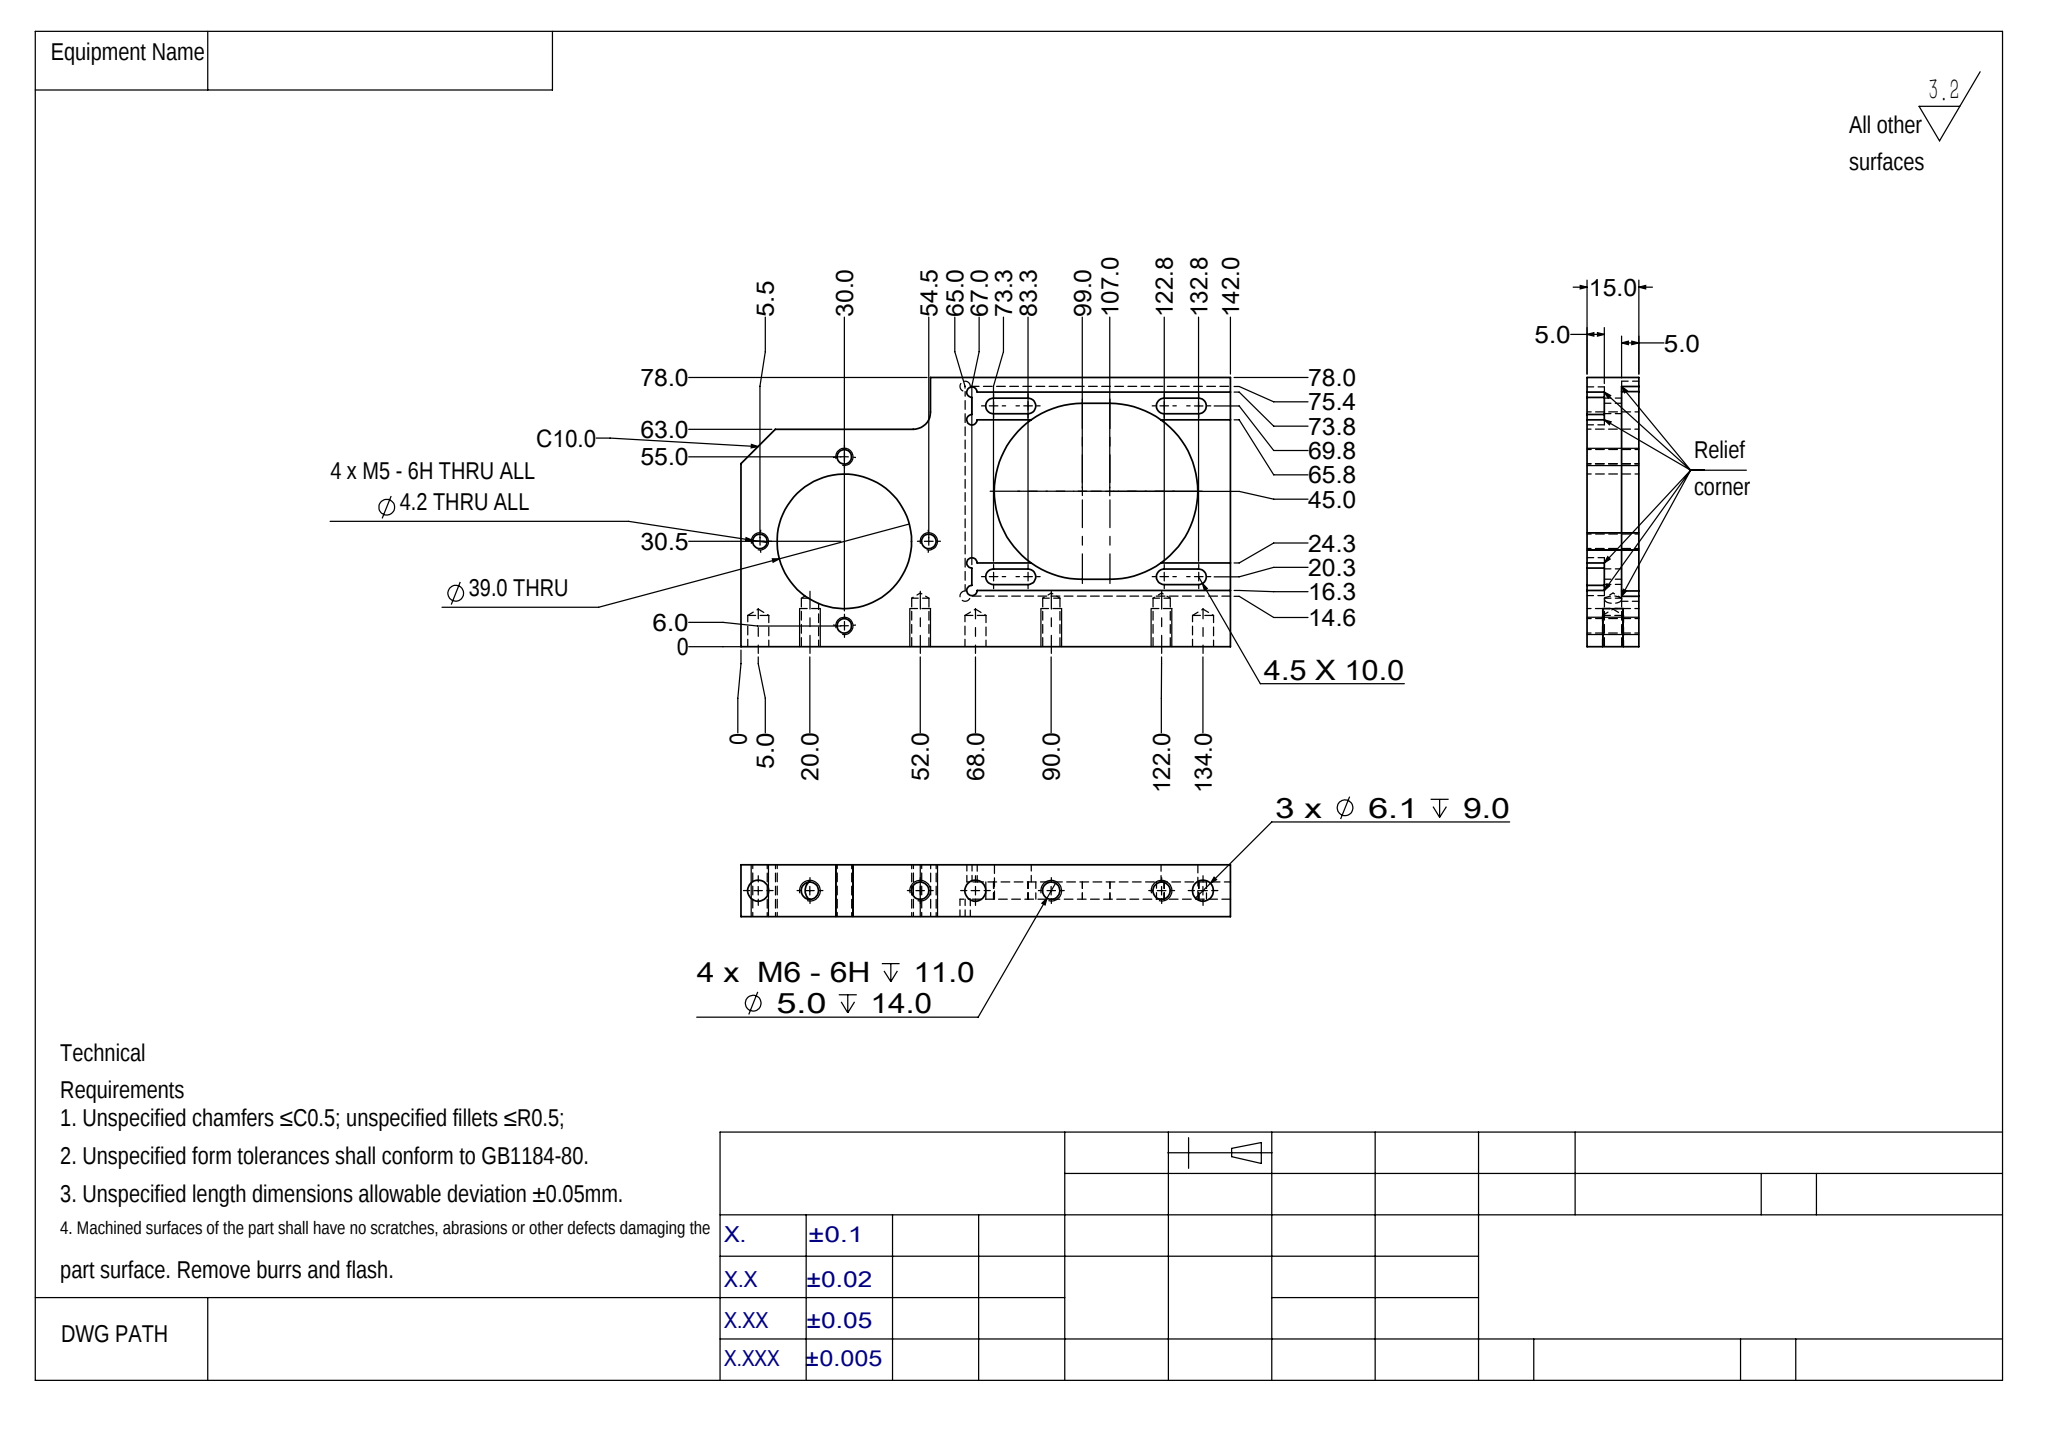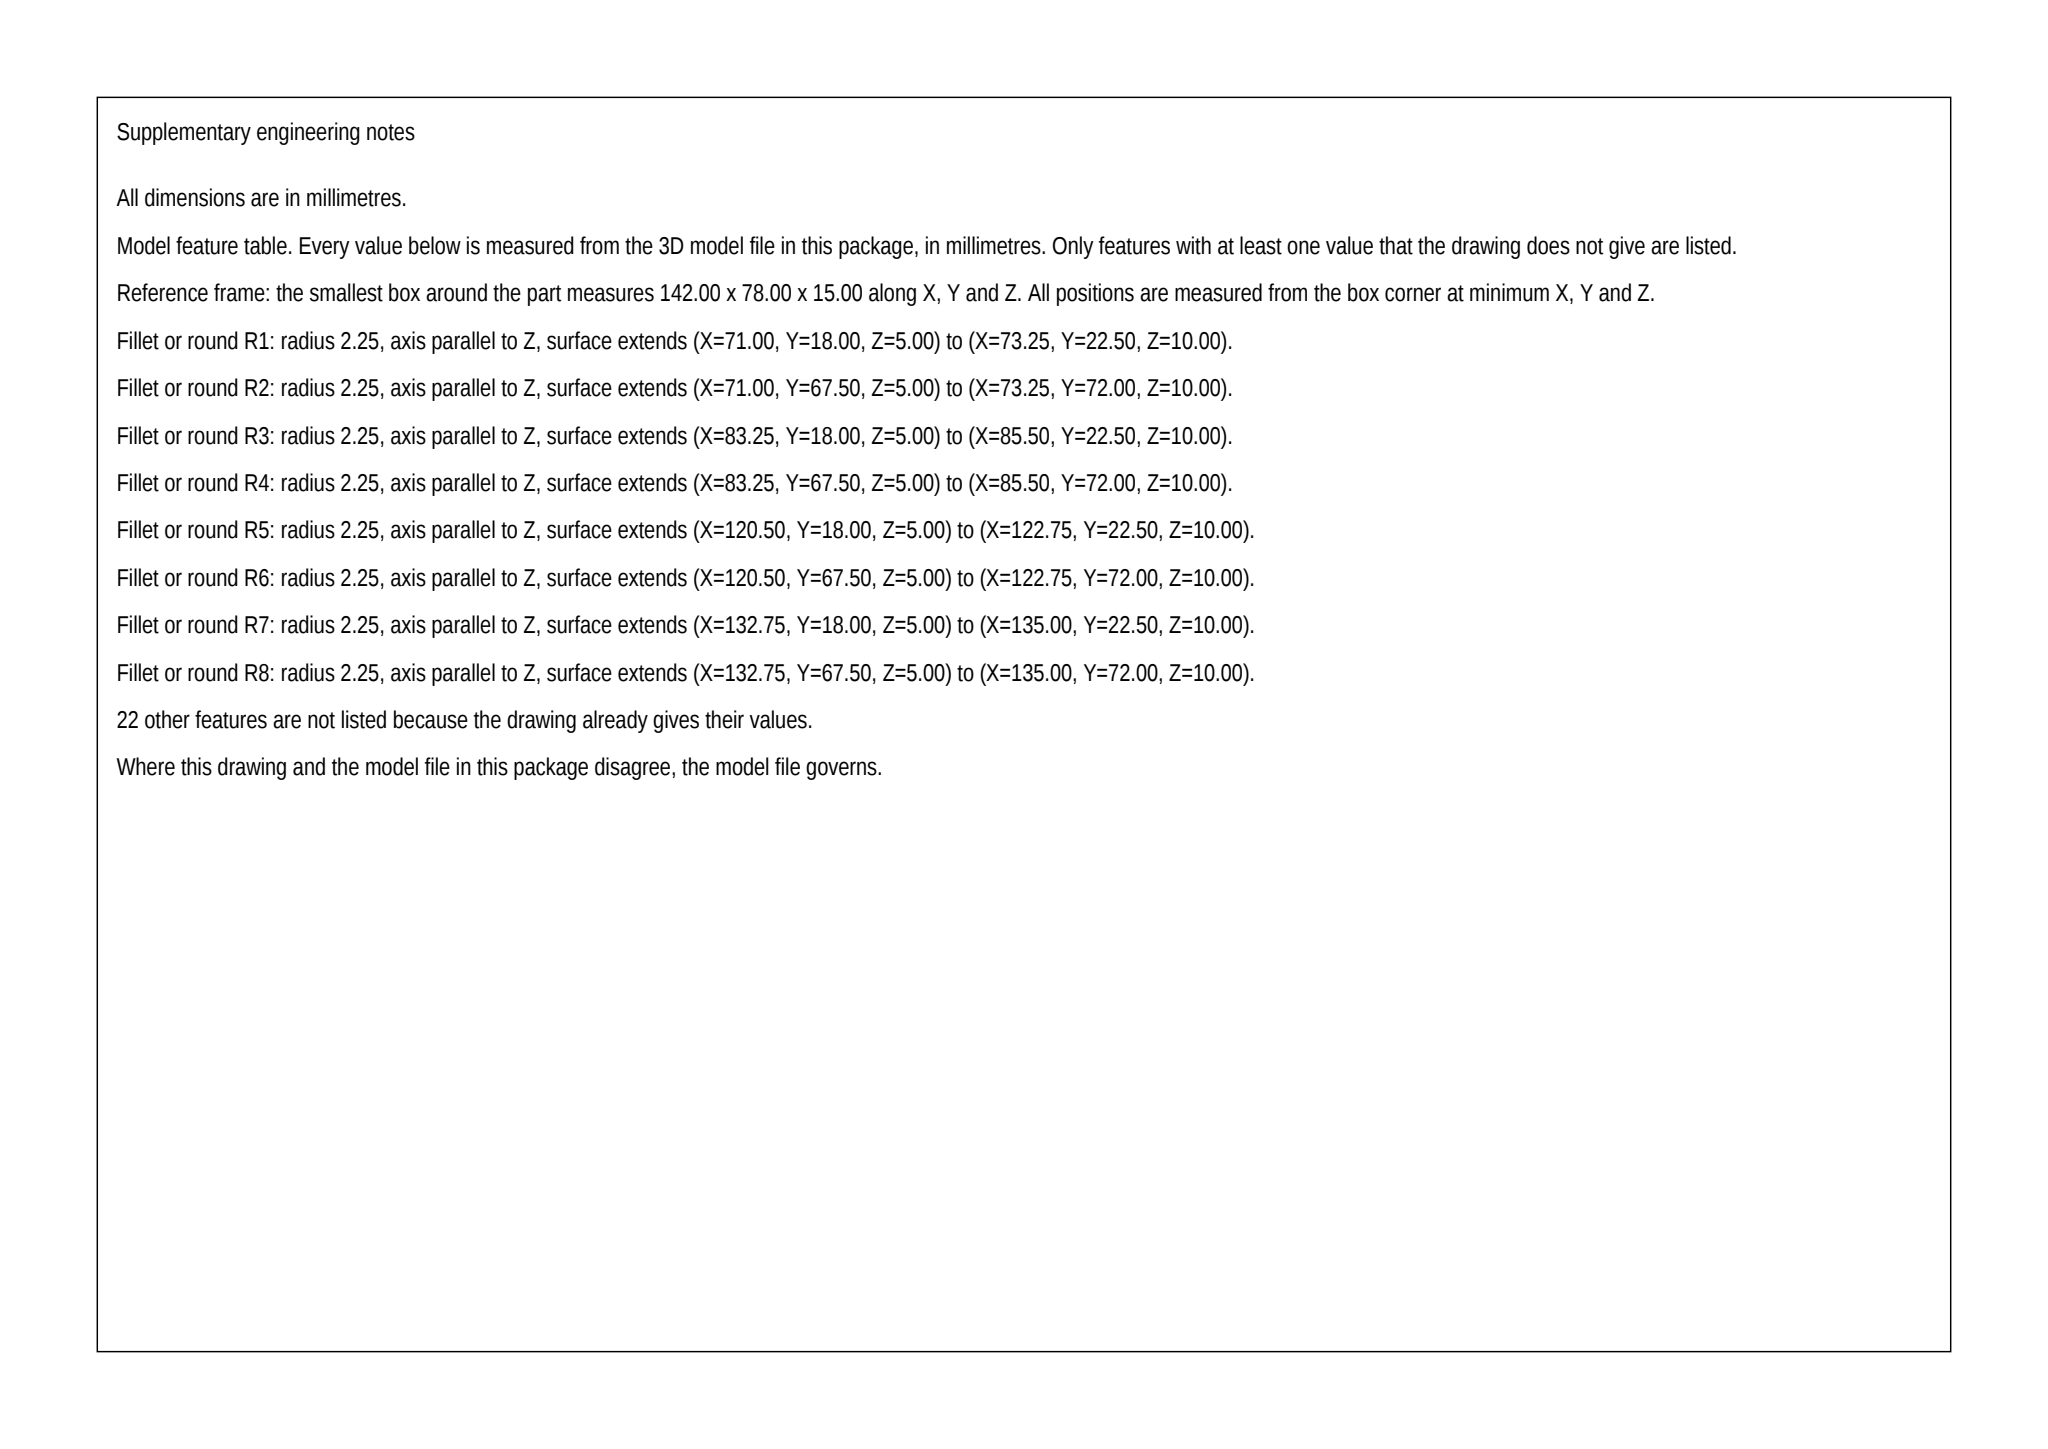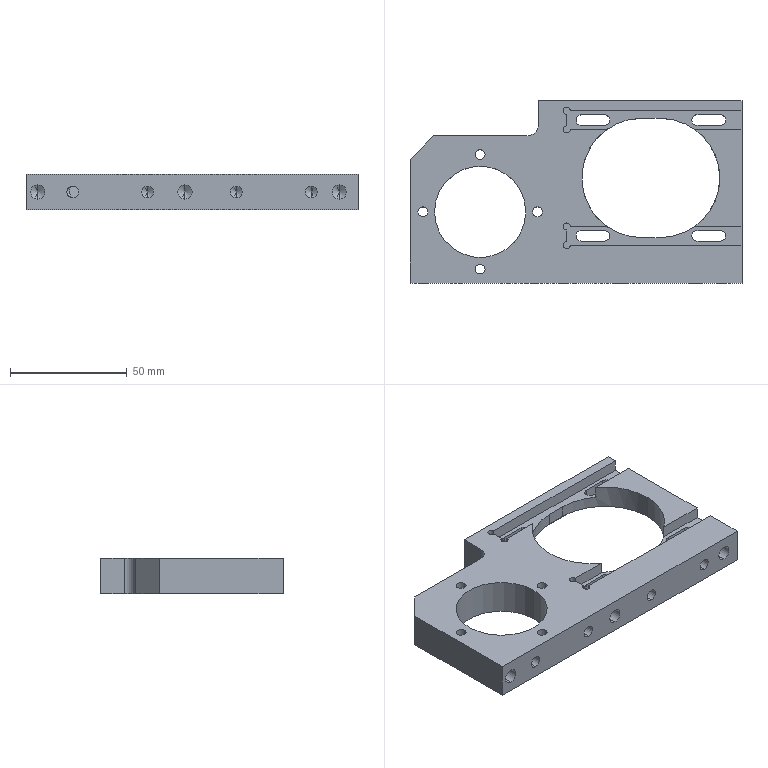Part | SolidWorks | mm | 1 solid | 95 faces | box 142 x 78 x 15 mm | volume 78424 mm3 | cylinder 48 | plane 34 | cone 13 | commonest cylinder face diameters 4.5 x12 5 x8 3 x8 4.2 x8 6.1 x6 51 x3 39 x2 10 x1
Drawing notes:
R25.5 OBROUND POCKET DP 10.0 FROM FRONT FACE (5.0 WEB REMAINS) | from the solid: Ø51 cyls at (99,45) & (107,45), axis z, length 10.0; z-planes at 5.0,15.0; bbox z=15.0
4X SLOT 4.5 X 10.0 DP 5.0 FROM BACK FACE, BREAKS INTO POCKET | from the solid: Ø4.5 z-cyls len 5.0 at x73.25/83.25 & x122.75/132.75, y20.25 & y69.75; z-plane 5.0
RELIEF SLOTS 2.0 WIDE DP 5.0 FROM BACK FACE, R1.5 CNRS | from the solid: Ø3.0 z-cyls len 5.0 at y14.6/16.25/24.25/65.75/73.75/75.4; y-planes 18/19.5/22.5 & 67.5/70.5/72
4X 4.5 X 10.0 SLOT, BACK FACE (OPP R25.5 POCKET) | from the solid: 4 slot pairs of Ø4.5 z-cyls len 5.0 at z0-5, pocket Ø51 at z5-15
VERT STEP FACE 55.0 FROM LEFT EDGE; R5.0 FILLET CL AT 50.0, 68.0 | from the solid: axis_plane x=55.0 (1); cylinder dia10.0 axis z at (50.0,68.0) = R5.0 internal fillet
build123d program:
from build123d import *

# Parameters (mm, degrees)
SKETCH1_W                      = 142
SKETCH1_H                      = 78
BOSS_EXTRUDE1_DEPTH            = 7.5
SKETCH2_R                      = 19.5
CUT_EXTRUDE1_DEPTH             = 83.383
SKETCH4_W                      = 77
SKETCH4_H                      = 60.8
CUT_EXTRUDE3_DEPTH             = 5
CUT_EXTRUDE4_DEPTH             = 83.383
M5_TAPPED_HOLE1_D              = 4.2
CIRPATTERN1_COUNT              = 4
SKETCH9_R                      = 1.5
CUT_EXTRUDE5_DEPTH             = 5
SKETCH10_W                     = 75
SKETCH10_H                     = 8
CUT_EXTRUDE6_DEPTH             = 5
LPATTERN1_COUNT                = 2
LPATTERN1_PITCH                = 49.5
SKETCH11_R                     = 1.5
CUT_EXTRUDE7_DEPTH             = 5
CUT_EXTRUDE8_DEPTH             = 10
LPATTERN2_COUNT                = 2
LPATTERN2_PITCH                = 49.5
LPATTERN2_COUNT_DIR2           = 2
LPATTERN2_PITCH_DIR2           = 49.5
SKETCH13_W                     = 55
SKETCH13_H                     = 15
CUT_EXTRUDE9_DEPTH             = 83.383
FILLET1_R                      = 5
M6_TAPPED_HOLE1_D              = 5
M6_TAPPED_HOLE1_DEPTH          = 14
M6_TAPPED_HOLE1_TIP            = 1.502
CHAMFER1_SIZE                  = 10
F_6_1_6_1_DIAMETER_HOLE1_D     = 6.1
F_6_1_6_1_DIAMETER_HOLE1_DEPTH = 9
F_6_1_6_1_DIAMETER_HOLE1_TIP   = 1.833


with BuildPart() as part:
    # Sketch1 → Boss-Extrude1 (new, symmetric)
    with BuildSketch(Plane.XY):
        Rectangle(SKETCH1_W, SKETCH1_H)
    extrude(amount=BOSS_EXTRUDE1_DEPTH, both=True)

    # Sketch2 → Cut-Extrude1 (cut, through all)
    with BuildSketch(Plane.XY.offset(7.5)):
        with Locations((-41, -8.5)):
            Circle(SKETCH2_R)
    extrude(amount=-CUT_EXTRUDE1_DEPTH, mode=Mode.SUBTRACT)

    # Sketch4 → Cut-Extrude3 (cut)
    with BuildSketch(Plane(origin=(0, 0, -7.5), x_dir=(-1, 0, 0), z_dir=(0, 0, -1))):
        with Locations((-32.5, 6)):
            Rectangle(SKETCH4_W, SKETCH4_H)
    extrude(amount=-CUT_EXTRUDE3_DEPTH, mode=Mode.SUBTRACT)

    # Sketch5 → Cut-Extrude4 (cut, through all)
    with BuildSketch(Plane.XY.offset(7.5)):
        with BuildLine():
            Line((36, -19.5), (28, -19.5))
            ThreePointArc((28, -19.5), (2.5, 6), (28, 31.5))
            Line((28, 31.5), (36, 31.5))
            ThreePointArc((36, 31.5), (61.5, 6), (36, -19.5))
        make_face()
    extrude(amount=-CUT_EXTRUDE4_DEPTH, mode=Mode.SUBTRACT)

    # M5 Tapped Hole1 (through all)
    with Locations(Plane(origin=(0, 0, -7.5), x_dir=(-1, 0, 0), z_dir=(0, 0, -1))):
        with Locations((41, -33)):
            m5_tapped_hole1 = Hole(M5_TAPPED_HOLE1_D / 2)

    # CirPattern1: M5 Tapped Hole1 ×4 about axis
    cirpattern1_axis = Axis((-41, -8.5, 0), (0, 0, 1))
    for i in range(1, CIRPATTERN1_COUNT):
        add(m5_tapped_hole1.rotate(cirpattern1_axis, i * 360 / CIRPATTERN1_COUNT), mode=Mode.SUBTRACT)

    # Sketch9 → Cut-Extrude5 (cut)
    with BuildSketch(Plane(origin=(0, 0, -7.5), x_dir=(-1, 0, 0), z_dir=(0, 0, -1))):
        with Locations((6, -24.4)):
            Circle(SKETCH9_R)
        with Locations((6, 36.4)):
            Circle(SKETCH9_R)
    extrude(amount=-CUT_EXTRUDE5_DEPTH, mode=Mode.SUBTRACT)

    # Sketch10 → Cut-Extrude6 (cut)
    with BuildSketch(Plane.XY.offset(7.5)):
        with Locations((33.5, 30.75)):
            Rectangle(SKETCH10_W, SKETCH10_H)
    cut_extrude6 = extrude(amount=-CUT_EXTRUDE6_DEPTH, mode=Mode.SUBTRACT)

    # LPattern1: Cut-Extrude6 ×2
    with Locations(*[(0, -i * LPATTERN1_PITCH, 0) for i in range(1, LPATTERN1_COUNT)]):
        add(cut_extrude6, mode=Mode.SUBTRACT)

    # Sketch11 → Cut-Extrude7 (cut)
    with BuildSketch(Plane.XY.offset(7.5)):
        with Locations((-4, 34.75)):
            Circle(SKETCH11_R)
        with Locations((-4, 26.75)):
            Circle(SKETCH11_R)
        with Locations((-4, -14.75)):
            Circle(SKETCH11_R)
        with Locations((-4, -22.75)):
            Circle(SKETCH11_R)
    extrude(amount=-CUT_EXTRUDE7_DEPTH, mode=Mode.SUBTRACT)

    # Sketch12 → Cut-Extrude8 (cut)
    with BuildSketch(Plane.XY.offset(2.5)):
        with BuildLine():
            Line((2.25, 33), (12.25, 33))
            ThreePointArc((12.25, 33), (14.5, 30.75), (12.25, 28.5))
            Line((12.25, 28.5), (2.25, 28.5))
            ThreePointArc((2.25, 28.5), (0, 30.75), (2.25, 33))
        make_face()
    cut_extrude8 = extrude(amount=-CUT_EXTRUDE8_DEPTH, mode=Mode.SUBTRACT)

    # LPattern2: Cut-Extrude8 2 × 2
    with Locations(*[(i * LPATTERN2_PITCH, -j * LPATTERN2_PITCH_DIR2, 0) for i in range(LPATTERN2_COUNT) for j in range(LPATTERN2_COUNT_DIR2) if (i, j) != (0, 0)]):
        add(cut_extrude8, mode=Mode.SUBTRACT)

    # Sketch13 → Cut-Extrude9 (cut, through all)
    with BuildSketch(Plane.XY.offset(7.5)):
        with Locations((-43.5, 31.5)):
            Rectangle(SKETCH13_W, SKETCH13_H)
    extrude(amount=-CUT_EXTRUDE9_DEPTH, mode=Mode.SUBTRACT)

    # Fillet1
    fillet1_edges = [part.edges().sort_by_distance(p)[0] for p in [
        (-16, 24, 0),
    ]]
    fillet(fillet1_edges, radius=FILLET1_R)

    # M6 Tapped Hole1
    with Locations(Plane(origin=(0, -39, 0), x_dir=(-1, 0, 0), z_dir=(0, -1, 0))):
        with Locations((19, 0), (51, 0), (-19, 0), (-51, 0)):
            Hole(M6_TAPPED_HOLE1_D / 2, depth=M6_TAPPED_HOLE1_DEPTH)
            with Locations((0, 0, -(M6_TAPPED_HOLE1_DEPTH + M6_TAPPED_HOLE1_TIP / 2))):  # 118° drill point
                Cone(0, M6_TAPPED_HOLE1_D / 2, M6_TAPPED_HOLE1_TIP, mode=Mode.SUBTRACT)

    # Chamfer1
    chamfer1_edges = [part.edges().sort_by_distance(p)[0] for p in [
        (-71, 24, 0),
    ]]
    chamfer(chamfer1_edges, length=CHAMFER1_SIZE)

    # 6.1 _6.1_ Diameter Hole1
    with Locations(Plane(origin=(0, -39, 0), x_dir=(-1, 0, 0), z_dir=(0, -1, 0))):
        with Locations((66, 0), (3, 0), (-63, 0)):
            Hole(F_6_1_6_1_DIAMETER_HOLE1_D / 2, depth=F_6_1_6_1_DIAMETER_HOLE1_DEPTH)
            with Locations((0, 0, -(F_6_1_6_1_DIAMETER_HOLE1_DEPTH + F_6_1_6_1_DIAMETER_HOLE1_TIP / 2))):  # 118° drill point
                Cone(0, F_6_1_6_1_DIAMETER_HOLE1_D / 2, F_6_1_6_1_DIAMETER_HOLE1_TIP, mode=Mode.SUBTRACT)


solid = part.part